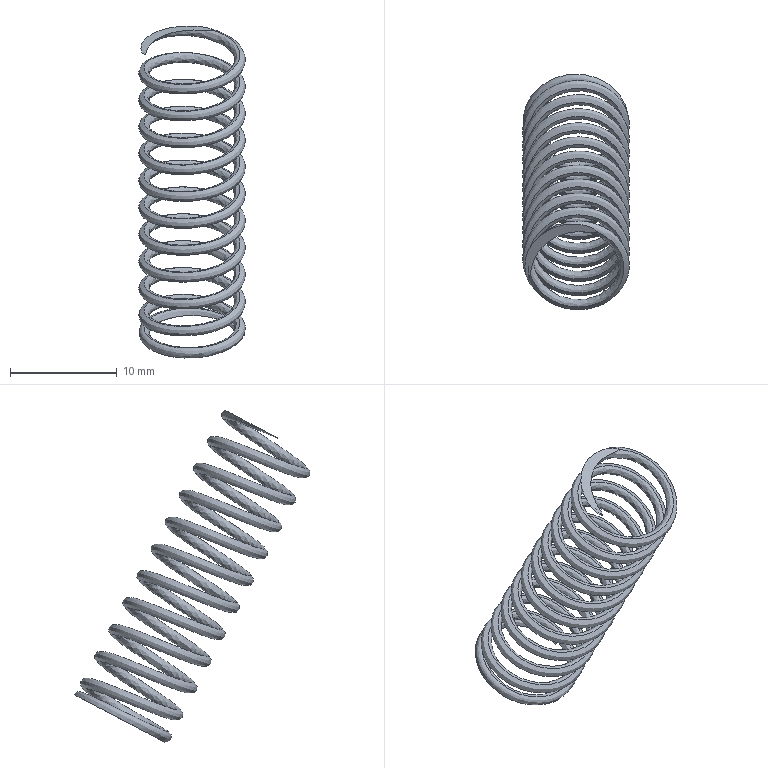Component | SolidWorks | Spring-2 | 1 solid | 5 faces | volume 246 mm3 | plane 3 | spline 2